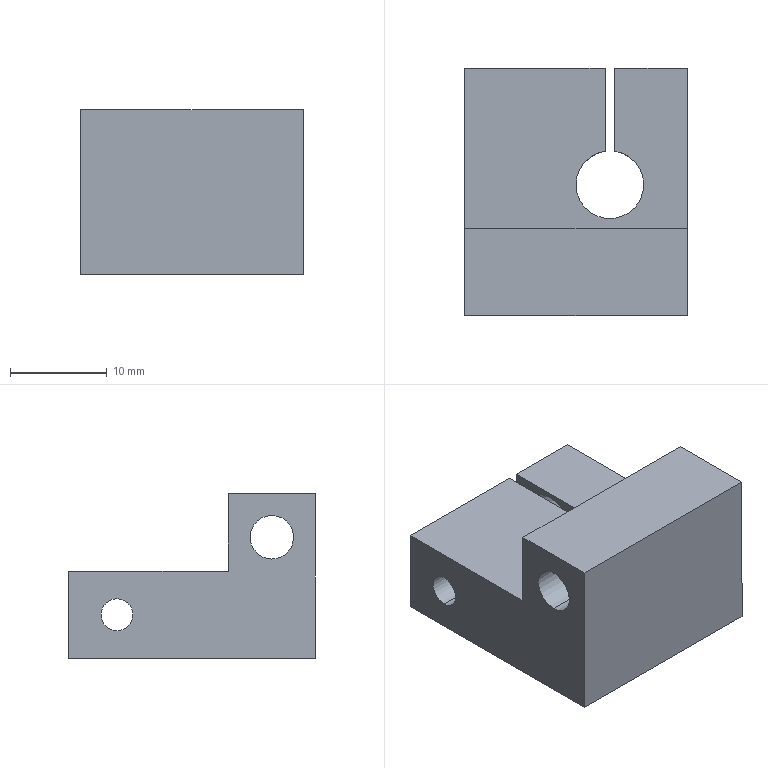Component | SolidWorks | AS-011-JG0137-1 | 1 solid | 26 faces | box 23 x 25.5 x 17 mm | volume 5301 mm3 | cylinder 13 | plane 13 | commonest cylinder face diameters 8 x4 7 x3 7.5 x2 4.5 x2 3.3 x2
STEP:
#1=COLOUR_RGB('',0.7922,0.8196,0.9333);
#2=FILL_AREA_STYLE_COLOUR('',#1);
#3=FILL_AREA_STYLE('',(#2));
#4=SURFACE_STYLE_FILL_AREA(#3);
#5=SURFACE_SIDE_STYLE('',(#4));
#6=SURFACE_STYLE_USAGE(.BOTH.,#5);
#7=PRESENTATION_STYLE_ASSIGNMENT((#6));
#8=CARTESIAN_POINT('',(-0.7283,-1.102,-1.476));
#9=VERTEX_POINT('',#8);
#10=CARTESIAN_POINT('',(-0.4528,-1.102,-1.476));
#11=VERTEX_POINT('',#10);
#12=CARTESIAN_POINT('',(-0.5906,-1.102,-1.476));
#13=DIRECTION('',(-0.,0.,1.));
#14=DIRECTION('',(1.,0.,0.));
#15=AXIS2_PLACEMENT_3D('',#12,#13,#14);
#16=CIRCLE('',#15,0.1378);
#17=EDGE_CURVE('',#9,#11,#16,.T.);
#18=ORIENTED_EDGE('',*,*,#17,.F.);
#19=CARTESIAN_POINT('',(-0.7283,-1.102,-1.122));
#20=VERTEX_POINT('',#19);
#21=CARTESIAN_POINT('',(-0.7283,-1.102,-1.476));
#22=DIRECTION('',(-0.,0.,1.));
#23=VECTOR('',#22,39.37);
#24=LINE('',#21,#23);
#25=EDGE_CURVE('',#9,#20,#24,.T.);
#26=ORIENTED_EDGE('',*,*,#25,.T.);
#27=CARTESIAN_POINT('',(-0.4528,-1.102,-1.122));
#28=VERTEX_POINT('',#27);
#29=CARTESIAN_POINT('',(-0.5906,-1.102,-1.122));
#30=DIRECTION('',(-0.,0.,1.));
#31=DIRECTION('',(1.,0.,0.));
#32=AXIS2_PLACEMENT_3D('',#29,#30,#31);
#33=CIRCLE('',#32,0.1378);
#34=EDGE_CURVE('',#20,#28,#33,.T.);
#35=ORIENTED_EDGE('',*,*,#34,.T.);
#36=CARTESIAN_POINT('',(-0.4528,-1.102,-1.476));
#37=DIRECTION('',(-0.,0.,1.));
#38=VECTOR('',#37,39.37);
#39=LINE('',#36,#38);
#40=EDGE_CURVE('',#11,#28,#39,.T.);
#41=ORIENTED_EDGE('',*,*,#40,.F.);
#42=EDGE_LOOP('',(#18,#26,#35,#41));
#43=FACE_OUTER_BOUND('',#42,.T.);
#44=CARTESIAN_POINT('',(-0.5906,-1.102,-1.476));
#45=DIRECTION('',(-0.,0.,1.));
#46=DIRECTION('',(1.,0.,0.));
#47=AXIS2_PLACEMENT_3D('',#44,#45,#46);
#48=CYLINDRICAL_SURFACE('',#47,0.1378);
#49=ADVANCED_FACE('',(#43),#48,.F.);
#50=CARTESIAN_POINT('',(-0.5709,-0.966,-1.476));
#51=VERTEX_POINT('',#50);
#52=CARTESIAN_POINT('',(-0.5906,-1.102,-1.476));
#53=DIRECTION('',(-0.,0.,1.));
#54=DIRECTION('',(1.,0.,0.));
#55=AXIS2_PLACEMENT_3D('',#52,#53,#54);
#56=CIRCLE('',#55,0.1378);
#57=EDGE_CURVE('',#11,#51,#56,.T.);
#58=ORIENTED_EDGE('',*,*,#57,.F.);
#59=ORIENTED_EDGE('',*,*,#40,.T.);
#60=CARTESIAN_POINT('',(-0.5709,-0.966,-1.122));
#61=VERTEX_POINT('',#60);
#62=CARTESIAN_POINT('',(-0.5906,-1.102,-1.122));
#63=DIRECTION('',(-0.,0.,1.));
#64=DIRECTION('',(1.,0.,0.));
#65=AXIS2_PLACEMENT_3D('',#62,#63,#64);
#66=CIRCLE('',#65,0.1378);
#67=EDGE_CURVE('',#28,#61,#66,.T.);
#68=ORIENTED_EDGE('',*,*,#67,.T.);
#69=CARTESIAN_POINT('',(-0.5709,-0.966,-1.226));
#70=VERTEX_POINT('',#69);
#71=CARTESIAN_POINT('',(-0.5709,-0.966,-1.476));
#72=DIRECTION('',(-0.,0.,1.));
#73=VECTOR('',#72,39.37);
#74=LINE('',#71,#73);
#75=EDGE_CURVE('',#70,#61,#74,.T.);
#76=ORIENTED_EDGE('',*,*,#75,.F.);
#77=CARTESIAN_POINT('',(-0.5709,-0.966,-1.373));
#78=VERTEX_POINT('',#77);
#79=CARTESIAN_POINT('',(-0.5709,-0.966,-1.373));
#80=CARTESIAN_POINT('',(-0.5629,-0.9671,-1.371));
#81=CARTESIAN_POINT('',(-0.5557,-0.9689,-1.367));
#82=CARTESIAN_POINT('',(-0.5426,-0.973,-1.358));
#83=CARTESIAN_POINT('',(-0.5371,-0.9752,-1.352));
#84=CARTESIAN_POINT('',(-0.5282,-0.9794,-1.339));
#85=CARTESIAN_POINT('',(-0.525,-0.9811,-1.331));
#86=CARTESIAN_POINT('',(-0.5206,-0.9836,-1.316));
#87=CARTESIAN_POINT('',(-0.5196,-0.9843,-1.307));
#88=CARTESIAN_POINT('',(-0.5196,-0.9843,-1.291));
#89=CARTESIAN_POINT('',(-0.5206,-0.9836,-1.283));
#90=CARTESIAN_POINT('',(-0.525,-0.9811,-1.267));
#91=CARTESIAN_POINT('',(-0.5282,-0.9794,-1.26));
#92=CARTESIAN_POINT('',(-0.5349,-0.9763,-1.25));
#93=CARTESIAN_POINT('',(-0.5374,-0.9752,-1.247));
#94=CARTESIAN_POINT('',(-0.5428,-0.9731,-1.241));
#95=CARTESIAN_POINT('',(-0.5458,-0.972,-1.238));
#96=CARTESIAN_POINT('',(-0.5523,-0.9699,-1.234));
#97=CARTESIAN_POINT('',(-0.5558,-0.969,-1.232));
#98=CARTESIAN_POINT('',(-0.5631,-0.9673,-1.228));
#99=CARTESIAN_POINT('',(-0.5669,-0.9666,-1.227));
#100=CARTESIAN_POINT('',(-0.5709,-0.966,-1.226));
#101=B_SPLINE_CURVE_WITH_KNOTS('',3,(#79,#80,#81,#82,#83,#84,#85,#86,#87,#88,#89,#90,#91,#92,#93,#94,#95,#96,#97,#98,#99,#100),.UNSPECIFIED.,.F.,.F.,(4,2,2,2,2,2,2,2,2,2,4),(0.,0.0006232,0.001246,0.00187,0.002493,0.003116,0.003739,0.004051,0.004363,0.004674,0.004986),.UNSPECIFIED.);
#102=EDGE_CURVE('',#78,#70,#101,.T.);
#103=ORIENTED_EDGE('',*,*,#102,.F.);
#104=CARTESIAN_POINT('',(-0.5709,-0.966,-1.476));
#105=DIRECTION('',(-0.,0.,1.));
#106=VECTOR('',#105,39.37);
#107=LINE('',#104,#106);
#108=EDGE_CURVE('',#51,#78,#107,.T.);
#109=ORIENTED_EDGE('',*,*,#108,.F.);
#110=EDGE_LOOP('',(#58,#59,#68,#76,#103,#109));
#111=FACE_OUTER_BOUND('',#110,.T.);
#112=CARTESIAN_POINT('',(-0.5906,-1.102,-1.476));
#113=DIRECTION('',(-0.,0.,1.));
#114=DIRECTION('',(1.,0.,0.));
#115=AXIS2_PLACEMENT_3D('',#112,#113,#114);
#116=CYLINDRICAL_SURFACE('',#115,0.1378);
#117=ADVANCED_FACE('',(#111),#116,.F.);
#118=CARTESIAN_POINT('',(-0.6693,-1.457,-0.8366));
#119=VERTEX_POINT('',#118);
#120=CARTESIAN_POINT('',(-0.6693,-1.457,-1.132));
#121=VERTEX_POINT('',#120);
#122=CARTESIAN_POINT('',(-0.6693,-1.457,-0.9843));
#123=DIRECTION('',(1.,0.,0.));
#124=DIRECTION('',(0.,0.,-1.));
#125=AXIS2_PLACEMENT_3D('',#122,#123,#124);
#126=CIRCLE('',#125,0.1476);
#127=EDGE_CURVE('',#119,#121,#126,.T.);
#128=ORIENTED_EDGE('',*,*,#127,.F.);
#129=CARTESIAN_POINT('',(-0.2756,-1.457,-0.8366));
#130=VERTEX_POINT('',#129);
#131=CARTESIAN_POINT('',(-0.6693,-1.457,-0.8366));
#132=DIRECTION('',(1.,0.,0.));
#133=VECTOR('',#132,39.37);
#134=LINE('',#131,#133);
#135=EDGE_CURVE('',#119,#130,#134,.T.);
#136=ORIENTED_EDGE('',*,*,#135,.T.);
#137=CARTESIAN_POINT('',(-0.2756,-1.457,-1.132));
#138=VERTEX_POINT('',#137);
#139=CARTESIAN_POINT('',(-0.2756,-1.457,-0.9843));
#140=DIRECTION('',(1.,0.,0.));
#141=DIRECTION('',(0.,0.,-1.));
#142=AXIS2_PLACEMENT_3D('',#139,#140,#141);
#143=CIRCLE('',#142,0.1476);
#144=EDGE_CURVE('',#130,#138,#143,.T.);
#145=ORIENTED_EDGE('',*,*,#144,.T.);
#146=CARTESIAN_POINT('',(-0.6693,-1.457,-1.132));
#147=DIRECTION('',(1.,0.,0.));
#148=VECTOR('',#147,39.37);
#149=LINE('',#146,#148);
#150=EDGE_CURVE('',#121,#138,#149,.T.);
#151=ORIENTED_EDGE('',*,*,#150,.F.);
#152=EDGE_LOOP('',(#128,#136,#145,#151));
#153=FACE_OUTER_BOUND('',#152,.T.);
#154=CARTESIAN_POINT('',(-0.6693,-1.457,-0.9843));
#155=DIRECTION('',(1.,0.,0.));
#156=DIRECTION('',(0.,0.,-1.));
#157=AXIS2_PLACEMENT_3D('',#154,#155,#156);
#158=CYLINDRICAL_SURFACE('',#157,0.1476);
#159=ADVANCED_FACE('',(#153),#158,.F.);
#160=CARTESIAN_POINT('',(-0.5709,-0.8268,-1.142));
#161=VERTEX_POINT('',#160);
#162=CARTESIAN_POINT('',(-0.5709,-0.8268,-1.299));
#163=DIRECTION('',(1.,0.,0.));
#164=DIRECTION('',(0.,0.,1.));
#165=AXIS2_PLACEMENT_3D('',#162,#163,#164);
#166=CIRCLE('',#165,0.1575);
#167=EDGE_CURVE('',#161,#70,#166,.T.);
#168=ORIENTED_EDGE('',*,*,#167,.F.);
#169=CARTESIAN_POINT('',(-0.2756,-0.8268,-1.142));
#170=VERTEX_POINT('',#169);
#171=CARTESIAN_POINT('',(-0.6693,-0.8268,-1.142));
#172=DIRECTION('',(1.,0.,0.));
#173=VECTOR('',#172,39.37);
#174=LINE('',#171,#173);
#175=EDGE_CURVE('',#161,#170,#174,.T.);
#176=ORIENTED_EDGE('',*,*,#175,.T.);
#177=CARTESIAN_POINT('',(-0.2756,-0.8268,-1.457));
#178=VERTEX_POINT('',#177);
#179=CARTESIAN_POINT('',(-0.2756,-0.8268,-1.299));
#180=DIRECTION('',(1.,0.,0.));
#181=DIRECTION('',(0.,-0.,-1.));
#182=AXIS2_PLACEMENT_3D('',#179,#180,#181);
#183=CIRCLE('',#182,0.1575);
#184=EDGE_CURVE('',#170,#178,#183,.T.);
#185=ORIENTED_EDGE('',*,*,#184,.T.);
#186=CARTESIAN_POINT('',(-0.5709,-0.8268,-1.457));
#187=VERTEX_POINT('',#186);
#188=CARTESIAN_POINT('',(-0.6693,-0.8268,-1.457));
#189=DIRECTION('',(1.,0.,0.));
#190=VECTOR('',#189,39.37);
#191=LINE('',#188,#190);
#192=EDGE_CURVE('',#187,#178,#191,.T.);
#193=ORIENTED_EDGE('',*,*,#192,.F.);
#194=CARTESIAN_POINT('',(-0.5709,-0.8268,-1.299));
#195=DIRECTION('',(1.,0.,0.));
#196=DIRECTION('',(0.,-0.,1.));
#197=AXIS2_PLACEMENT_3D('',#194,#195,#196);
#198=CIRCLE('',#197,0.1575);
#199=EDGE_CURVE('',#78,#187,#198,.T.);
#200=ORIENTED_EDGE('',*,*,#199,.F.);
#201=ORIENTED_EDGE('',*,*,#102,.T.);
#202=EDGE_LOOP('',(#168,#176,#185,#193,#200,#201));
#203=FACE_OUTER_BOUND('',#202,.T.);
#204=CARTESIAN_POINT('',(-0.6693,-0.8268,-1.299));
#205=DIRECTION('',(1.,0.,0.));
#206=DIRECTION('',(0.,-0.,-1.));
#207=AXIS2_PLACEMENT_3D('',#204,#205,#206);
#208=CYLINDRICAL_SURFACE('',#207,0.1575);
#209=ADVANCED_FACE('',(#203),#208,.F.);
#210=CARTESIAN_POINT('',(-1.181,-1.457,-0.8957));
#211=VERTEX_POINT('',#210);
#212=CARTESIAN_POINT('',(-1.181,-1.457,-1.073));
#213=VERTEX_POINT('',#212);
#214=CARTESIAN_POINT('',(-1.181,-1.457,-0.9843));
#215=DIRECTION('',(1.,0.,0.));
#216=DIRECTION('',(0.,0.,-1.));
#217=AXIS2_PLACEMENT_3D('',#214,#215,#216);
#218=CIRCLE('',#217,0.08858);
#219=EDGE_CURVE('',#211,#213,#218,.T.);
#220=ORIENTED_EDGE('',*,*,#219,.F.);
#221=CARTESIAN_POINT('',(-0.6693,-1.457,-0.8957));
#222=VERTEX_POINT('',#221);
#223=CARTESIAN_POINT('',(-1.181,-1.457,-0.8957));
#224=DIRECTION('',(1.,0.,0.));
#225=VECTOR('',#224,39.37);
#226=LINE('',#223,#225);
#227=EDGE_CURVE('',#211,#222,#226,.T.);
#228=ORIENTED_EDGE('',*,*,#227,.T.);
#229=CARTESIAN_POINT('',(-0.6693,-1.457,-1.073));
#230=VERTEX_POINT('',#229);
#231=CARTESIAN_POINT('',(-0.6693,-1.457,-0.9843));
#232=DIRECTION('',(1.,0.,0.));
#233=DIRECTION('',(0.,0.,-1.));
#234=AXIS2_PLACEMENT_3D('',#231,#232,#233);
#235=CIRCLE('',#234,0.08858);
#236=EDGE_CURVE('',#222,#230,#235,.T.);
#237=ORIENTED_EDGE('',*,*,#236,.T.);
#238=CARTESIAN_POINT('',(-1.181,-1.457,-1.073));
#239=DIRECTION('',(1.,0.,0.));
#240=VECTOR('',#239,39.37);
#241=LINE('',#238,#240);
#242=EDGE_CURVE('',#213,#230,#241,.T.);
#243=ORIENTED_EDGE('',*,*,#242,.F.);
#244=EDGE_LOOP('',(#220,#228,#237,#243));
#245=FACE_OUTER_BOUND('',#244,.T.);
#246=CARTESIAN_POINT('',(-1.181,-1.457,-0.9843));
#247=DIRECTION('',(1.,0.,0.));
#248=DIRECTION('',(0.,0.,-1.));
#249=AXIS2_PLACEMENT_3D('',#246,#247,#248);
#250=CYLINDRICAL_SURFACE('',#249,0.08858);
#251=ADVANCED_FACE('',(#245),#250,.F.);
#252=CARTESIAN_POINT('',(-1.181,-0.8268,-1.234));
#253=VERTEX_POINT('',#252);
#254=CARTESIAN_POINT('',(-1.181,-0.8268,-1.364));
#255=VERTEX_POINT('',#254);
#256=CARTESIAN_POINT('',(-1.181,-0.8268,-1.299));
#257=DIRECTION('',(1.,0.,0.));
#258=DIRECTION('',(0.,0.,-1.));
#259=AXIS2_PLACEMENT_3D('',#256,#257,#258);
#260=CIRCLE('',#259,0.06496);
#261=EDGE_CURVE('',#253,#255,#260,.T.);
#262=ORIENTED_EDGE('',*,*,#261,.F.);
#263=CARTESIAN_POINT('',(-0.6693,-0.8268,-1.234));
#264=VERTEX_POINT('',#263);
#265=CARTESIAN_POINT('',(-1.181,-0.8268,-1.234));
#266=DIRECTION('',(1.,0.,0.));
#267=VECTOR('',#266,39.37);
#268=LINE('',#265,#267);
#269=EDGE_CURVE('',#253,#264,#268,.T.);
#270=ORIENTED_EDGE('',*,*,#269,.T.);
#271=CARTESIAN_POINT('',(-0.6693,-0.8268,-1.364));
#272=VERTEX_POINT('',#271);
#273=CARTESIAN_POINT('',(-0.6693,-0.8268,-1.299));
#274=DIRECTION('',(1.,0.,0.));
#275=DIRECTION('',(0.,0.,-1.));
#276=AXIS2_PLACEMENT_3D('',#273,#274,#275);
#277=CIRCLE('',#276,0.06496);
#278=EDGE_CURVE('',#264,#272,#277,.T.);
#279=ORIENTED_EDGE('',*,*,#278,.T.);
#280=CARTESIAN_POINT('',(-1.181,-0.8268,-1.364));
#281=DIRECTION('',(1.,0.,0.));
#282=VECTOR('',#281,39.37);
#283=LINE('',#280,#282);
#284=EDGE_CURVE('',#255,#272,#283,.T.);
#285=ORIENTED_EDGE('',*,*,#284,.F.);
#286=EDGE_LOOP('',(#262,#270,#279,#285));
#287=FACE_OUTER_BOUND('',#286,.T.);
#288=CARTESIAN_POINT('',(-1.181,-0.8268,-1.299));
#289=DIRECTION('',(1.,0.,0.));
#290=DIRECTION('',(0.,0.,-1.));
#291=AXIS2_PLACEMENT_3D('',#288,#289,#290);
#292=CYLINDRICAL_SURFACE('',#291,0.06496);
#293=ADVANCED_FACE('',(#287),#292,.F.);
#294=CARTESIAN_POINT('',(-0.6693,-0.8268,-1.142));
#295=VERTEX_POINT('',#294);
#296=CARTESIAN_POINT('',(-0.6693,-0.8268,-1.457));
#297=VERTEX_POINT('',#296);
#298=CARTESIAN_POINT('',(-0.6693,-0.8268,-1.299));
#299=DIRECTION('',(1.,0.,0.));
#300=DIRECTION('',(0.,-0.,-1.));
#301=AXIS2_PLACEMENT_3D('',#298,#299,#300);
#302=CIRCLE('',#301,0.1575);
#303=EDGE_CURVE('',#295,#297,#302,.T.);
#304=ORIENTED_EDGE('',*,*,#303,.F.);
#305=CARTESIAN_POINT('',(-0.6102,-0.8268,-1.142));
#306=VERTEX_POINT('',#305);
#307=CARTESIAN_POINT('',(-0.6693,-0.8268,-1.142));
#308=DIRECTION('',(1.,0.,0.));
#309=VECTOR('',#308,39.37);
#310=LINE('',#307,#309);
#311=EDGE_CURVE('',#295,#306,#310,.T.);
#312=ORIENTED_EDGE('',*,*,#311,.T.);
#313=CARTESIAN_POINT('',(-0.6102,-0.966,-1.226));
#314=VERTEX_POINT('',#313);
#315=CARTESIAN_POINT('',(-0.6102,-0.8268,-1.299));
#316=DIRECTION('',(1.,0.,0.));
#317=DIRECTION('',(0.,0.,1.));
#318=AXIS2_PLACEMENT_3D('',#315,#316,#317);
#319=CIRCLE('',#318,0.1575);
#320=EDGE_CURVE('',#306,#314,#319,.T.);
#321=ORIENTED_EDGE('',*,*,#320,.T.);
#322=CARTESIAN_POINT('',(-0.6102,-0.966,-1.373));
#323=VERTEX_POINT('',#322);
#324=CARTESIAN_POINT('',(-0.6102,-0.966,-1.226));
#325=CARTESIAN_POINT('',(-0.6182,-0.9671,-1.228));
#326=CARTESIAN_POINT('',(-0.6254,-0.9689,-1.231));
#327=CARTESIAN_POINT('',(-0.6385,-0.973,-1.241));
#328=CARTESIAN_POINT('',(-0.644,-0.9752,-1.246));
#329=CARTESIAN_POINT('',(-0.6529,-0.9794,-1.26));
#330=CARTESIAN_POINT('',(-0.6561,-0.9811,-1.267));
#331=CARTESIAN_POINT('',(-0.6605,-0.9836,-1.283));
#332=CARTESIAN_POINT('',(-0.6615,-0.9843,-1.291));
#333=CARTESIAN_POINT('',(-0.6615,-0.9843,-1.308));
#334=CARTESIAN_POINT('',(-0.6605,-0.9836,-1.316));
#335=CARTESIAN_POINT('',(-0.6561,-0.9811,-1.331));
#336=CARTESIAN_POINT('',(-0.6529,-0.9794,-1.339));
#337=CARTESIAN_POINT('',(-0.6463,-0.9763,-1.349));
#338=CARTESIAN_POINT('',(-0.6437,-0.9752,-1.352));
#339=CARTESIAN_POINT('',(-0.6383,-0.9731,-1.358));
#340=CARTESIAN_POINT('',(-0.6353,-0.972,-1.36));
#341=CARTESIAN_POINT('',(-0.6288,-0.9699,-1.365));
#342=CARTESIAN_POINT('',(-0.6253,-0.969,-1.367));
#343=CARTESIAN_POINT('',(-0.618,-0.9673,-1.37));
#344=CARTESIAN_POINT('',(-0.6142,-0.9666,-1.372));
#345=CARTESIAN_POINT('',(-0.6102,-0.966,-1.373));
#346=B_SPLINE_CURVE_WITH_KNOTS('',3,(#324,#325,#326,#327,#328,#329,#330,#331,#332,#333,#334,#335,#336,#337,#338,#339,#340,#341,#342,#343,#344,#345),.UNSPECIFIED.,.F.,.F.,(4,2,2,2,2,2,2,2,2,2,4),(0.,0.0006232,0.001246,0.00187,0.002493,0.003116,0.003739,0.004051,0.004363,0.004674,0.004986),.UNSPECIFIED.);
#347=EDGE_CURVE('',#314,#323,#346,.T.);
#348=ORIENTED_EDGE('',*,*,#347,.T.);
#349=CARTESIAN_POINT('',(-0.6102,-0.8268,-1.457));
#350=VERTEX_POINT('',#349);
#351=CARTESIAN_POINT('',(-0.6102,-0.8268,-1.299));
#352=DIRECTION('',(1.,0.,0.));
#353=DIRECTION('',(0.,-0.,1.));
#354=AXIS2_PLACEMENT_3D('',#351,#352,#353);
#355=CIRCLE('',#354,0.1575);
#356=EDGE_CURVE('',#323,#350,#355,.T.);
#357=ORIENTED_EDGE('',*,*,#356,.T.);
#358=CARTESIAN_POINT('',(-0.6693,-0.8268,-1.457));
#359=DIRECTION('',(1.,0.,0.));
#360=VECTOR('',#359,39.37);
#361=LINE('',#358,#360);
#362=EDGE_CURVE('',#297,#350,#361,.T.);
#363=ORIENTED_EDGE('',*,*,#362,.F.);
#364=EDGE_LOOP('',(#304,#312,#321,#348,#357,#363));
#365=FACE_OUTER_BOUND('',#364,.T.);
#366=CARTESIAN_POINT('',(-0.6693,-0.8268,-1.299));
#367=DIRECTION('',(1.,0.,0.));
#368=DIRECTION('',(0.,-0.,-1.));
#369=AXIS2_PLACEMENT_3D('',#366,#367,#368);
#370=CYLINDRICAL_SURFACE('',#369,0.1575);
#371=ADVANCED_FACE('',(#365),#370,.F.);
#372=CARTESIAN_POINT('',(-0.5709,-0.6299,-1.476));
#373=VERTEX_POINT('',#372);
#374=CARTESIAN_POINT('',(-0.5709,-0.6299,-1.122));
#375=VERTEX_POINT('',#374);
#376=CARTESIAN_POINT('',(-0.5709,-0.6299,-1.476));
#377=DIRECTION('',(-0.,0.,1.));
#378=VECTOR('',#377,39.37);
#379=LINE('',#376,#378);
#380=EDGE_CURVE('',#373,#375,#379,.T.);
#381=ORIENTED_EDGE('',*,*,#380,.T.);
#382=CARTESIAN_POINT('',(-0.2756,-0.6299,-1.122));
#383=VERTEX_POINT('',#382);
#384=CARTESIAN_POINT('',(-1.181,-0.6299,-1.122));
#385=DIRECTION('',(1.,0.,0.));
#386=VECTOR('',#385,39.37);
#387=LINE('',#384,#386);
#388=EDGE_CURVE('',#375,#383,#387,.T.);
#389=ORIENTED_EDGE('',*,*,#388,.T.);
#390=CARTESIAN_POINT('',(-0.2756,-0.6299,-1.476));
#391=VERTEX_POINT('',#390);
#392=CARTESIAN_POINT('',(-0.2756,-0.6299,-1.122));
#393=DIRECTION('',(0.,-0.,-1.));
#394=VECTOR('',#393,39.37);
#395=LINE('',#392,#394);
#396=EDGE_CURVE('',#383,#391,#395,.T.);
#397=ORIENTED_EDGE('',*,*,#396,.T.);
#398=CARTESIAN_POINT('',(-1.181,-0.6299,-1.476));
#399=DIRECTION('',(1.,0.,0.));
#400=VECTOR('',#399,39.37);
#401=LINE('',#398,#400);
#402=EDGE_CURVE('',#373,#391,#401,.T.);
#403=ORIENTED_EDGE('',*,*,#402,.F.);
#404=EDGE_LOOP('',(#381,#389,#397,#403));
#405=FACE_OUTER_BOUND('',#404,.T.);
#406=CARTESIAN_POINT('',(-1.181,-0.6299,-1.122));
#407=DIRECTION('',(0.,-1.,0.));
#408=DIRECTION('',(-1.,-0.,-0.));
#409=AXIS2_PLACEMENT_3D('',#406,#407,#408);
#410=PLANE('',#409);
#411=ADVANCED_FACE('',(#405),#410,.F.);
#412=ORIENTED_EDGE('',*,*,#311,.F.);
#413=CARTESIAN_POINT('',(-0.6693,-0.8268,-1.299));
#414=DIRECTION('',(1.,0.,0.));
#415=DIRECTION('',(0.,-0.,-1.));
#416=AXIS2_PLACEMENT_3D('',#413,#414,#415);
#417=CIRCLE('',#416,0.1575);
#418=EDGE_CURVE('',#297,#295,#417,.T.);
#419=ORIENTED_EDGE('',*,*,#418,.F.);
#420=ORIENTED_EDGE('',*,*,#362,.T.);
#421=CARTESIAN_POINT('',(-0.6102,-0.8268,-1.299));
#422=DIRECTION('',(1.,0.,0.));
#423=DIRECTION('',(0.,0.,1.));
#424=AXIS2_PLACEMENT_3D('',#421,#422,#423);
#425=CIRCLE('',#424,0.1575);
#426=EDGE_CURVE('',#350,#306,#425,.T.);
#427=ORIENTED_EDGE('',*,*,#426,.T.);
#428=EDGE_LOOP('',(#412,#419,#420,#427));
#429=FACE_OUTER_BOUND('',#428,.T.);
#430=CARTESIAN_POINT('',(-0.6693,-0.8268,-1.299));
#431=DIRECTION('',(1.,0.,0.));
#432=DIRECTION('',(0.,-0.,-1.));
#433=AXIS2_PLACEMENT_3D('',#430,#431,#432);
#434=CYLINDRICAL_SURFACE('',#433,0.1575);
#435=ADVANCED_FACE('',(#429),#434,.F.);
#436=ORIENTED_EDGE('',*,*,#269,.F.);
#437=CARTESIAN_POINT('',(-1.181,-0.8268,-1.299));
#438=DIRECTION('',(1.,0.,0.));
#439=DIRECTION('',(0.,0.,-1.));
#440=AXIS2_PLACEMENT_3D('',#437,#438,#439);
#441=CIRCLE('',#440,0.06496);
#442=EDGE_CURVE('',#255,#253,#441,.T.);
#443=ORIENTED_EDGE('',*,*,#442,.F.);
#444=ORIENTED_EDGE('',*,*,#284,.T.);
#445=CARTESIAN_POINT('',(-0.6693,-0.8268,-1.299));
#446=DIRECTION('',(1.,0.,0.));
#447=DIRECTION('',(0.,0.,-1.));
#448=AXIS2_PLACEMENT_3D('',#445,#446,#447);
#449=CIRCLE('',#448,0.06496);
#450=EDGE_CURVE('',#272,#264,#449,.T.);
#451=ORIENTED_EDGE('',*,*,#450,.T.);
#452=EDGE_LOOP('',(#436,#443,#444,#451));
#453=FACE_OUTER_BOUND('',#452,.T.);
#454=CARTESIAN_POINT('',(-1.181,-0.8268,-1.299));
#455=DIRECTION('',(1.,0.,0.));
#456=DIRECTION('',(0.,0.,-1.));
#457=AXIS2_PLACEMENT_3D('',#454,#455,#456);
#458=CYLINDRICAL_SURFACE('',#457,0.06496);
#459=ADVANCED_FACE('',(#453),#458,.F.);
#460=ORIENTED_EDGE('',*,*,#227,.F.);
#461=CARTESIAN_POINT('',(-1.181,-1.457,-0.9843));
#462=DIRECTION('',(1.,0.,0.));
#463=DIRECTION('',(0.,0.,-1.));
#464=AXIS2_PLACEMENT_3D('',#461,#462,#463);
#465=CIRCLE('',#464,0.08858);
#466=EDGE_CURVE('',#213,#211,#465,.T.);
#467=ORIENTED_EDGE('',*,*,#466,.F.);
#468=ORIENTED_EDGE('',*,*,#242,.T.);
#469=CARTESIAN_POINT('',(-0.6693,-1.457,-0.9843));
#470=DIRECTION('',(1.,0.,0.));
#471=DIRECTION('',(0.,0.,-1.));
#472=AXIS2_PLACEMENT_3D('',#469,#470,#471);
#473=CIRCLE('',#472,0.08858);
#474=EDGE_CURVE('',#230,#222,#473,.T.);
#475=ORIENTED_EDGE('',*,*,#474,.T.);
#476=EDGE_LOOP('',(#460,#467,#468,#475));
#477=FACE_OUTER_BOUND('',#476,.T.);
#478=CARTESIAN_POINT('',(-1.181,-1.457,-0.9843));
#479=DIRECTION('',(1.,0.,0.));
#480=DIRECTION('',(0.,0.,-1.));
#481=AXIS2_PLACEMENT_3D('',#478,#479,#480);
#482=CYLINDRICAL_SURFACE('',#481,0.08858);
#483=ADVANCED_FACE('',(#477),#482,.F.);
#484=CARTESIAN_POINT('',(-1.181,-0.6299,-1.476));
#485=VERTEX_POINT('',#484);
#486=CARTESIAN_POINT('',(-0.6102,-0.6299,-1.476));
#487=VERTEX_POINT('',#486);
#488=CARTESIAN_POINT('',(-1.181,-0.6299,-1.476));
#489=DIRECTION('',(1.,0.,0.));
#490=VECTOR('',#489,39.37);
#491=LINE('',#488,#490);
#492=EDGE_CURVE('',#485,#487,#491,.T.);
#493=ORIENTED_EDGE('',*,*,#492,.T.);
#494=CARTESIAN_POINT('',(-0.6102,-0.966,-1.476));
#495=VERTEX_POINT('',#494);
#496=CARTESIAN_POINT('',(-0.6102,-0.6299,-1.476));
#497=DIRECTION('',(0.,-1.,0.));
#498=VECTOR('',#497,39.37);
#499=LINE('',#496,#498);
#500=EDGE_CURVE('',#487,#495,#499,.T.);
#501=ORIENTED_EDGE('',*,*,#500,.T.);
#502=CARTESIAN_POINT('',(-0.5906,-1.102,-1.476));
#503=DIRECTION('',(-0.,0.,1.));
#504=DIRECTION('',(1.,0.,0.));
#505=AXIS2_PLACEMENT_3D('',#502,#503,#504);
#506=CIRCLE('',#505,0.1378);
#507=EDGE_CURVE('',#495,#9,#506,.T.);
#508=ORIENTED_EDGE('',*,*,#507,.T.);
#509=ORIENTED_EDGE('',*,*,#17,.T.);
#510=ORIENTED_EDGE('',*,*,#57,.T.);
#511=CARTESIAN_POINT('',(-0.5709,-0.6299,-1.476));
#512=DIRECTION('',(0.,-1.,0.));
#513=VECTOR('',#512,39.37);
#514=LINE('',#511,#513);
#515=EDGE_CURVE('',#373,#51,#514,.T.);
#516=ORIENTED_EDGE('',*,*,#515,.F.);
#517=ORIENTED_EDGE('',*,*,#402,.T.);
#518=CARTESIAN_POINT('',(-0.2756,-1.634,-1.476));
#519=VERTEX_POINT('',#518);
#520=CARTESIAN_POINT('',(-0.2756,-0.6299,-1.476));
#521=DIRECTION('',(0.,-1.,0.));
#522=VECTOR('',#521,39.37);
#523=LINE('',#520,#522);
#524=EDGE_CURVE('',#391,#519,#523,.T.);
#525=ORIENTED_EDGE('',*,*,#524,.T.);
#526=CARTESIAN_POINT('',(-1.181,-1.634,-1.476));
#527=VERTEX_POINT('',#526);
#528=CARTESIAN_POINT('',(-1.181,-1.634,-1.476));
#529=DIRECTION('',(1.,0.,0.));
#530=VECTOR('',#529,39.37);
#531=LINE('',#528,#530);
#532=EDGE_CURVE('',#527,#519,#531,.T.);
#533=ORIENTED_EDGE('',*,*,#532,.F.);
#534=CARTESIAN_POINT('',(-1.181,-0.6299,-1.476));
#535=DIRECTION('',(0.,-1.,0.));
#536=VECTOR('',#535,39.37);
#537=LINE('',#534,#536);
#538=EDGE_CURVE('',#485,#527,#537,.T.);
#539=ORIENTED_EDGE('',*,*,#538,.F.);
#540=EDGE_LOOP('',(#493,#501,#508,#509,#510,#516,#517,#525,#533,#539));
#541=FACE_OUTER_BOUND('',#540,.T.);
#542=CARTESIAN_POINT('',(-1.181,-0.6299,-1.476));
#543=DIRECTION('',(-0.,0.,1.));
#544=DIRECTION('',(1.,0.,0.));
#545=AXIS2_PLACEMENT_3D('',#542,#543,#544);
#546=PLANE('',#545);
#547=ADVANCED_FACE('',(#541),#546,.F.);
#548=CARTESIAN_POINT('',(-0.2756,-1.634,-0.8071));
#549=VERTEX_POINT('',#548);
#550=CARTESIAN_POINT('',(-0.2756,-1.634,-0.8071));
#551=DIRECTION('',(0.,-0.,-1.));
#552=VECTOR('',#551,39.37);
#553=LINE('',#550,#552);
#554=EDGE_CURVE('',#549,#519,#553,.T.);
#555=ORIENTED_EDGE('',*,*,#554,.F.);
#556=CARTESIAN_POINT('',(-1.181,-1.634,-0.8071));
#557=VERTEX_POINT('',#556);
#558=CARTESIAN_POINT('',(-1.181,-1.634,-0.8071));
#559=DIRECTION('',(1.,0.,0.));
#560=VECTOR('',#559,39.37);
#561=LINE('',#558,#560);
#562=EDGE_CURVE('',#557,#549,#561,.T.);
#563=ORIENTED_EDGE('',*,*,#562,.F.);
#564=CARTESIAN_POINT('',(-1.181,-1.634,-0.8071));
#565=DIRECTION('',(0.,-0.,-1.));
#566=VECTOR('',#565,39.37);
#567=LINE('',#564,#566);
#568=EDGE_CURVE('',#557,#527,#567,.T.);
#569=ORIENTED_EDGE('',*,*,#568,.T.);
#570=ORIENTED_EDGE('',*,*,#532,.T.);
#571=EDGE_LOOP('',(#555,#563,#569,#570));
#572=FACE_OUTER_BOUND('',#571,.T.);
#573=CARTESIAN_POINT('',(-1.181,-1.634,-0.8071));
#574=DIRECTION('',(0.,-1.,0.));
#575=DIRECTION('',(-1.,-0.,-0.));
#576=AXIS2_PLACEMENT_3D('',#573,#574,#575);
#577=PLANE('',#576);
#578=ADVANCED_FACE('',(#572),#577,.T.);
#579=CARTESIAN_POINT('',(-0.2756,-1.28,-0.8071));
#580=VERTEX_POINT('',#579);
#581=CARTESIAN_POINT('',(-0.2756,-1.28,-0.8071));
#582=DIRECTION('',(0.,-1.,0.));
#583=VECTOR('',#582,39.37);
#584=LINE('',#581,#583);
#585=EDGE_CURVE('',#580,#549,#584,.T.);
#586=ORIENTED_EDGE('',*,*,#585,.F.);
#587=CARTESIAN_POINT('',(-1.181,-1.28,-0.8071));
#588=VERTEX_POINT('',#587);
#589=CARTESIAN_POINT('',(-1.181,-1.28,-0.8071));
#590=DIRECTION('',(1.,0.,0.));
#591=VECTOR('',#590,39.37);
#592=LINE('',#589,#591);
#593=EDGE_CURVE('',#588,#580,#592,.T.);
#594=ORIENTED_EDGE('',*,*,#593,.F.);
#595=CARTESIAN_POINT('',(-1.181,-1.28,-0.8071));
#596=DIRECTION('',(0.,-1.,0.));
#597=VECTOR('',#596,39.37);
#598=LINE('',#595,#597);
#599=EDGE_CURVE('',#588,#557,#598,.T.);
#600=ORIENTED_EDGE('',*,*,#599,.T.);
#601=ORIENTED_EDGE('',*,*,#562,.T.);
#602=EDGE_LOOP('',(#586,#594,#600,#601));
#603=FACE_OUTER_BOUND('',#602,.T.);
#604=CARTESIAN_POINT('',(-1.181,-1.28,-0.8071));
#605=DIRECTION('',(-0.,0.,1.));
#606=DIRECTION('',(1.,0.,0.));
#607=AXIS2_PLACEMENT_3D('',#604,#605,#606);
#608=PLANE('',#607);
#609=ADVANCED_FACE('',(#603),#608,.T.);
#610=CARTESIAN_POINT('',(-0.2756,-1.28,-1.122));
#611=VERTEX_POINT('',#610);
#612=CARTESIAN_POINT('',(-0.2756,-1.28,-0.8071));
#613=DIRECTION('',(0.,-0.,-1.));
#614=VECTOR('',#613,39.37);
#615=LINE('',#612,#614);
#616=EDGE_CURVE('',#580,#611,#615,.T.);
#617=ORIENTED_EDGE('',*,*,#616,.T.);
#618=CARTESIAN_POINT('',(-1.181,-1.28,-1.122));
#619=VERTEX_POINT('',#618);
#620=CARTESIAN_POINT('',(-1.181,-1.28,-1.122));
#621=DIRECTION('',(1.,0.,0.));
#622=VECTOR('',#621,39.37);
#623=LINE('',#620,#622);
#624=EDGE_CURVE('',#619,#611,#623,.T.);
#625=ORIENTED_EDGE('',*,*,#624,.F.);
#626=CARTESIAN_POINT('',(-1.181,-1.28,-0.8071));
#627=DIRECTION('',(0.,-0.,-1.));
#628=VECTOR('',#627,39.37);
#629=LINE('',#626,#628);
#630=EDGE_CURVE('',#588,#619,#629,.T.);
#631=ORIENTED_EDGE('',*,*,#630,.F.);
#632=ORIENTED_EDGE('',*,*,#593,.T.);
#633=EDGE_LOOP('',(#617,#625,#631,#632));
#634=FACE_OUTER_BOUND('',#633,.T.);
#635=CARTESIAN_POINT('',(-1.181,-1.28,-0.8071));
#636=DIRECTION('',(0.,-1.,0.));
#637=DIRECTION('',(-1.,-0.,-0.));
#638=AXIS2_PLACEMENT_3D('',#635,#636,#637);
#639=PLANE('',#638);
#640=ADVANCED_FACE('',(#634),#639,.F.);
#641=CARTESIAN_POINT('',(-0.6102,-0.6299,-1.122));
#642=VERTEX_POINT('',#641);
#643=CARTESIAN_POINT('',(-0.6102,-0.966,-1.122));
#644=VERTEX_POINT('',#643);
#645=CARTESIAN_POINT('',(-0.6102,-0.6299,-1.122));
#646=DIRECTION('',(0.,-1.,0.));
#647=VECTOR('',#646,39.37);
#648=LINE('',#645,#647);
#649=EDGE_CURVE('',#642,#644,#648,.T.);
#650=ORIENTED_EDGE('',*,*,#649,.F.);
#651=CARTESIAN_POINT('',(-1.181,-0.6299,-1.122));
#652=VERTEX_POINT('',#651);
#653=CARTESIAN_POINT('',(-1.181,-0.6299,-1.122));
#654=DIRECTION('',(1.,0.,0.));
#655=VECTOR('',#654,39.37);
#656=LINE('',#653,#655);
#657=EDGE_CURVE('',#652,#642,#656,.T.);
#658=ORIENTED_EDGE('',*,*,#657,.F.);
#659=CARTESIAN_POINT('',(-1.181,-0.6299,-1.122));
#660=DIRECTION('',(0.,-1.,0.));
#661=VECTOR('',#660,39.37);
#662=LINE('',#659,#661);
#663=EDGE_CURVE('',#652,#619,#662,.T.);
#664=ORIENTED_EDGE('',*,*,#663,.T.);
#665=ORIENTED_EDGE('',*,*,#624,.T.);
#666=CARTESIAN_POINT('',(-0.2756,-0.6299,-1.122));
#667=DIRECTION('',(0.,-1.,0.));
#668=VECTOR('',#667,39.37);
#669=LINE('',#666,#668);
#670=EDGE_CURVE('',#383,#611,#669,.T.);
#671=ORIENTED_EDGE('',*,*,#670,.F.);
#672=ORIENTED_EDGE('',*,*,#388,.F.);
#673=CARTESIAN_POINT('',(-0.5709,-0.6299,-1.122));
#674=DIRECTION('',(0.,-1.,0.));
#675=VECTOR('',#674,39.37);
#676=LINE('',#673,#675);
#677=EDGE_CURVE('',#375,#61,#676,.T.);
#678=ORIENTED_EDGE('',*,*,#677,.T.);
#679=ORIENTED_EDGE('',*,*,#67,.F.);
#680=ORIENTED_EDGE('',*,*,#34,.F.);
#681=CARTESIAN_POINT('',(-0.5906,-1.102,-1.122));
#682=DIRECTION('',(-0.,0.,1.));
#683=DIRECTION('',(1.,0.,0.));
#684=AXIS2_PLACEMENT_3D('',#681,#682,#683);
#685=CIRCLE('',#684,0.1378);
#686=EDGE_CURVE('',#644,#20,#685,.T.);
#687=ORIENTED_EDGE('',*,*,#686,.F.);
#688=EDGE_LOOP('',(#650,#658,#664,#665,#671,#672,#678,#679,#680,#687));
#689=FACE_OUTER_BOUND('',#688,.T.);
#690=CARTESIAN_POINT('',(-1.181,-0.6299,-1.122));
#691=DIRECTION('',(-0.,0.,1.));
#692=DIRECTION('',(1.,0.,0.));
#693=AXIS2_PLACEMENT_3D('',#690,#691,#692);
#694=PLANE('',#693);
#695=ADVANCED_FACE('',(#689),#694,.T.);
#696=ORIENTED_EDGE('',*,*,#657,.T.);
#697=CARTESIAN_POINT('',(-0.6102,-0.6299,-1.476));
#698=DIRECTION('',(-0.,0.,1.));
#699=VECTOR('',#698,39.37);
#700=LINE('',#697,#699);
#701=EDGE_CURVE('',#487,#642,#700,.T.);
#702=ORIENTED_EDGE('',*,*,#701,.F.);
#703=ORIENTED_EDGE('',*,*,#492,.F.);
#704=CARTESIAN_POINT('',(-1.181,-0.6299,-1.122));
#705=DIRECTION('',(0.,-0.,-1.));
#706=VECTOR('',#705,39.37);
#707=LINE('',#704,#706);
#708=EDGE_CURVE('',#652,#485,#707,.T.);
#709=ORIENTED_EDGE('',*,*,#708,.F.);
#710=EDGE_LOOP('',(#696,#702,#703,#709));
#711=FACE_OUTER_BOUND('',#710,.T.);
#712=CARTESIAN_POINT('',(-1.181,-0.6299,-1.122));
#713=DIRECTION('',(0.,-1.,0.));
#714=DIRECTION('',(-1.,-0.,-0.));
#715=AXIS2_PLACEMENT_3D('',#712,#713,#714);
#716=PLANE('',#715);
#717=ADVANCED_FACE('',(#711),#716,.F.);
#718=ORIENTED_EDGE('',*,*,#466,.T.);
#719=ORIENTED_EDGE('',*,*,#219,.T.);
#720=EDGE_LOOP('',(#718,#719));
#721=FACE_BOUND('',#720,.T.);
#722=ORIENTED_EDGE('',*,*,#442,.T.);
#723=ORIENTED_EDGE('',*,*,#261,.T.);
#724=EDGE_LOOP('',(#722,#723));
#725=FACE_BOUND('',#724,.T.);
#726=ORIENTED_EDGE('',*,*,#538,.T.);
#727=ORIENTED_EDGE('',*,*,#568,.F.);
#728=ORIENTED_EDGE('',*,*,#599,.F.);
#729=ORIENTED_EDGE('',*,*,#630,.T.);
#730=ORIENTED_EDGE('',*,*,#663,.F.);
#731=ORIENTED_EDGE('',*,*,#708,.T.);
#732=EDGE_LOOP('',(#726,#727,#728,#729,#730,#731));
#733=FACE_OUTER_BOUND('',#732,.T.);
#734=CARTESIAN_POINT('',(-1.181,-1.634,-1.476));
#735=DIRECTION('',(1.,0.,0.));
#736=DIRECTION('',(0.,-0.,-1.));
#737=AXIS2_PLACEMENT_3D('',#734,#735,#736);
#738=PLANE('',#737);
#739=ADVANCED_FACE('',(#721,#725,#733),#738,.F.);
#740=CARTESIAN_POINT('',(-0.2756,-1.457,-0.9843));
#741=DIRECTION('',(1.,0.,0.));
#742=DIRECTION('',(0.,0.,-1.));
#743=AXIS2_PLACEMENT_3D('',#740,#741,#742);
#744=CIRCLE('',#743,0.1476);
#745=EDGE_CURVE('',#138,#130,#744,.T.);
#746=ORIENTED_EDGE('',*,*,#745,.F.);
#747=ORIENTED_EDGE('',*,*,#144,.F.);
#748=EDGE_LOOP('',(#746,#747));
#749=FACE_BOUND('',#748,.T.);
#750=CARTESIAN_POINT('',(-0.2756,-0.8268,-1.299));
#751=DIRECTION('',(1.,0.,0.));
#752=DIRECTION('',(0.,-0.,-1.));
#753=AXIS2_PLACEMENT_3D('',#750,#751,#752);
#754=CIRCLE('',#753,0.1575);
#755=EDGE_CURVE('',#178,#170,#754,.T.);
#756=ORIENTED_EDGE('',*,*,#755,.F.);
#757=ORIENTED_EDGE('',*,*,#184,.F.);
#758=EDGE_LOOP('',(#756,#757));
#759=FACE_BOUND('',#758,.T.);
#760=ORIENTED_EDGE('',*,*,#524,.F.);
#761=ORIENTED_EDGE('',*,*,#396,.F.);
#762=ORIENTED_EDGE('',*,*,#670,.T.);
#763=ORIENTED_EDGE('',*,*,#616,.F.);
#764=ORIENTED_EDGE('',*,*,#585,.T.);
#765=ORIENTED_EDGE('',*,*,#554,.T.);
#766=EDGE_LOOP('',(#760,#761,#762,#763,#764,#765));
#767=FACE_OUTER_BOUND('',#766,.T.);
#768=CARTESIAN_POINT('',(-0.2756,-1.634,-1.476));
#769=DIRECTION('',(1.,0.,0.));
#770=DIRECTION('',(0.,-0.,-1.));
#771=AXIS2_PLACEMENT_3D('',#768,#769,#770);
#772=PLANE('',#771);
#773=ADVANCED_FACE('',(#749,#759,#767),#772,.T.);
#774=ORIENTED_EDGE('',*,*,#175,.F.);
#775=CARTESIAN_POINT('',(-0.5709,-0.8268,-1.299));
#776=DIRECTION('',(1.,0.,0.));
#777=DIRECTION('',(0.,0.,1.));
#778=AXIS2_PLACEMENT_3D('',#775,#776,#777);
#779=CIRCLE('',#778,0.1575);
#780=EDGE_CURVE('',#187,#161,#779,.T.);
#781=ORIENTED_EDGE('',*,*,#780,.F.);
#782=ORIENTED_EDGE('',*,*,#192,.T.);
#783=ORIENTED_EDGE('',*,*,#755,.T.);
#784=EDGE_LOOP('',(#774,#781,#782,#783));
#785=FACE_OUTER_BOUND('',#784,.T.);
#786=CARTESIAN_POINT('',(-0.6693,-0.8268,-1.299));
#787=DIRECTION('',(1.,0.,0.));
#788=DIRECTION('',(0.,-0.,-1.));
#789=AXIS2_PLACEMENT_3D('',#786,#787,#788);
#790=CYLINDRICAL_SURFACE('',#789,0.1575);
#791=ADVANCED_FACE('',(#785),#790,.F.);
#792=ORIENTED_EDGE('',*,*,#418,.T.);
#793=ORIENTED_EDGE('',*,*,#303,.T.);
#794=EDGE_LOOP('',(#792,#793));
#795=FACE_OUTER_BOUND('',#794,.T.);
#796=ORIENTED_EDGE('',*,*,#450,.F.);
#797=ORIENTED_EDGE('',*,*,#278,.F.);
#798=EDGE_LOOP('',(#796,#797));
#799=FACE_BOUND('',#798,.T.);
#800=CARTESIAN_POINT('',(-0.6693,-1.634,-1.476));
#801=DIRECTION('',(1.,0.,0.));
#802=DIRECTION('',(0.,-0.,-1.));
#803=AXIS2_PLACEMENT_3D('',#800,#801,#802);
#804=PLANE('',#803);
#805=ADVANCED_FACE('',(#795,#799),#804,.T.);
#806=ORIENTED_EDGE('',*,*,#135,.F.);
#807=CARTESIAN_POINT('',(-0.6693,-1.457,-0.9843));
#808=DIRECTION('',(1.,0.,0.));
#809=DIRECTION('',(0.,0.,-1.));
#810=AXIS2_PLACEMENT_3D('',#807,#808,#809);
#811=CIRCLE('',#810,0.1476);
#812=EDGE_CURVE('',#121,#119,#811,.T.);
#813=ORIENTED_EDGE('',*,*,#812,.F.);
#814=ORIENTED_EDGE('',*,*,#150,.T.);
#815=ORIENTED_EDGE('',*,*,#745,.T.);
#816=EDGE_LOOP('',(#806,#813,#814,#815));
#817=FACE_OUTER_BOUND('',#816,.T.);
#818=CARTESIAN_POINT('',(-0.6693,-1.457,-0.9843));
#819=DIRECTION('',(1.,0.,0.));
#820=DIRECTION('',(0.,0.,-1.));
#821=AXIS2_PLACEMENT_3D('',#818,#819,#820);
#822=CYLINDRICAL_SURFACE('',#821,0.1476);
#823=ADVANCED_FACE('',(#817),#822,.F.);
#824=ORIENTED_EDGE('',*,*,#474,.F.);
#825=ORIENTED_EDGE('',*,*,#236,.F.);
#826=EDGE_LOOP('',(#824,#825));
#827=FACE_BOUND('',#826,.T.);
#828=ORIENTED_EDGE('',*,*,#812,.T.);
#829=ORIENTED_EDGE('',*,*,#127,.T.);
#830=EDGE_LOOP('',(#828,#829));
#831=FACE_OUTER_BOUND('',#830,.T.);
#832=CARTESIAN_POINT('',(-0.6693,-1.634,-1.476));
#833=DIRECTION('',(1.,0.,0.));
#834=DIRECTION('',(0.,-0.,-1.));
#835=AXIS2_PLACEMENT_3D('',#832,#833,#834);
#836=PLANE('',#835);
#837=ADVANCED_FACE('',(#827,#831),#836,.T.);
#838=ORIENTED_EDGE('',*,*,#649,.T.);
#839=CARTESIAN_POINT('',(-0.6102,-0.966,-1.476));
#840=DIRECTION('',(-0.,0.,1.));
#841=VECTOR('',#840,39.37);
#842=LINE('',#839,#841);
#843=EDGE_CURVE('',#314,#644,#842,.T.);
#844=ORIENTED_EDGE('',*,*,#843,.F.);
#845=ORIENTED_EDGE('',*,*,#320,.F.);
#846=ORIENTED_EDGE('',*,*,#426,.F.);
#847=ORIENTED_EDGE('',*,*,#356,.F.);
#848=CARTESIAN_POINT('',(-0.6102,-0.966,-1.476));
#849=DIRECTION('',(-0.,0.,1.));
#850=VECTOR('',#849,39.37);
#851=LINE('',#848,#850);
#852=EDGE_CURVE('',#495,#323,#851,.T.);
#853=ORIENTED_EDGE('',*,*,#852,.F.);
#854=ORIENTED_EDGE('',*,*,#500,.F.);
#855=ORIENTED_EDGE('',*,*,#701,.T.);
#856=EDGE_LOOP('',(#838,#844,#845,#846,#847,#853,#854,#855));
#857=FACE_OUTER_BOUND('',#856,.T.);
#858=CARTESIAN_POINT('',(-0.6102,-0.6299,-1.476));
#859=DIRECTION('',(-1.,-0.,-0.));
#860=DIRECTION('',(-0.,0.,1.));
#861=AXIS2_PLACEMENT_3D('',#858,#859,#860);
#862=PLANE('',#861);
#863=ADVANCED_FACE('',(#857),#862,.F.);
#864=ORIENTED_EDGE('',*,*,#25,.F.);
#865=ORIENTED_EDGE('',*,*,#507,.F.);
#866=ORIENTED_EDGE('',*,*,#852,.T.);
#867=ORIENTED_EDGE('',*,*,#347,.F.);
#868=ORIENTED_EDGE('',*,*,#843,.T.);
#869=ORIENTED_EDGE('',*,*,#686,.T.);
#870=EDGE_LOOP('',(#864,#865,#866,#867,#868,#869));
#871=FACE_OUTER_BOUND('',#870,.T.);
#872=CARTESIAN_POINT('',(-0.5906,-1.102,-1.476));
#873=DIRECTION('',(-0.,0.,1.));
#874=DIRECTION('',(1.,0.,0.));
#875=AXIS2_PLACEMENT_3D('',#872,#873,#874);
#876=CYLINDRICAL_SURFACE('',#875,0.1378);
#877=ADVANCED_FACE('',(#871),#876,.F.);
#878=ORIENTED_EDGE('',*,*,#380,.F.);
#879=ORIENTED_EDGE('',*,*,#515,.T.);
#880=ORIENTED_EDGE('',*,*,#108,.T.);
#881=ORIENTED_EDGE('',*,*,#199,.T.);
#882=ORIENTED_EDGE('',*,*,#780,.T.);
#883=ORIENTED_EDGE('',*,*,#167,.T.);
#884=ORIENTED_EDGE('',*,*,#75,.T.);
#885=ORIENTED_EDGE('',*,*,#677,.F.);
#886=EDGE_LOOP('',(#878,#879,#880,#881,#882,#883,#884,#885));
#887=FACE_OUTER_BOUND('',#886,.T.);
#888=CARTESIAN_POINT('',(-0.5709,-0.6299,-1.476));
#889=DIRECTION('',(-1.,-0.,-0.));
#890=DIRECTION('',(-0.,0.,1.));
#891=AXIS2_PLACEMENT_3D('',#888,#889,#890);
#892=PLANE('',#891);
#893=ADVANCED_FACE('',(#887),#892,.T.);
#894=CLOSED_SHELL('',(#49,#117,#159,#209,#251,#293,#371,#411,#435,#459,#483,#547,#578,#609,#640,#695,#717,#739,#773,#791,#805,#823,#837,#863,#877,#893));
#895=MANIFOLD_SOLID_BREP('',#894);
#896=STYLED_ITEM('',(#7),#895);
#897=PRESENTATION_LAYER_ASSIGNMENT('','',(#896));
#898=(LENGTH_UNIT()NAMED_UNIT(*)SI_UNIT($,.METRE.));
#899=LENGTH_MEASURE_WITH_UNIT(LENGTH_MEASURE(0.0254),#898);
#900=DIMENSIONAL_EXPONENTS(1.,0.,0.,0.,0.,0.,0.);
#901=(CONVERSION_BASED_UNIT('',#899)LENGTH_UNIT()NAMED_UNIT(#900));
#902=UNCERTAINTY_MEASURE_WITH_UNIT(LENGTH_MEASURE(0.00001),#901,'','');
#903=(NAMED_UNIT(*)PLANE_ANGLE_UNIT()SI_UNIT($,.RADIAN.));
#904=(NAMED_UNIT(*)SI_UNIT($,.STERADIAN.)SOLID_ANGLE_UNIT());
#905=(GEOMETRIC_REPRESENTATION_CONTEXT(3)GLOBAL_UNCERTAINTY_ASSIGNED_CONTEXT((#902))GLOBAL_UNIT_ASSIGNED_CONTEXT((#901,#903,#904))REPRESENTATION_CONTEXT('',''));
#906=MECHANICAL_DESIGN_GEOMETRIC_PRESENTATION_REPRESENTATION('',(#896),#905);
#907=CARTESIAN_POINT('',(0.,0.,0.));
#908=DIRECTION('',(0.,0.,1.));
#909=DIRECTION('',(1.,0.,0.));
#910=AXIS2_PLACEMENT_3D('',#907,#908,#909);
#911=(LENGTH_UNIT()NAMED_UNIT(*)SI_UNIT($,.METRE.));
#912=LENGTH_MEASURE_WITH_UNIT(LENGTH_MEASURE(0.0254),#911);
#913=DIMENSIONAL_EXPONENTS(1.,0.,0.,0.,0.,0.,0.);
#914=(CONVERSION_BASED_UNIT('',#912)LENGTH_UNIT()NAMED_UNIT(#913));
#915=UNCERTAINTY_MEASURE_WITH_UNIT(LENGTH_MEASURE(0.00001),#914,'','');
#916=(NAMED_UNIT(*)PLANE_ANGLE_UNIT()SI_UNIT($,.RADIAN.));
#917=(NAMED_UNIT(*)SI_UNIT($,.STERADIAN.)SOLID_ANGLE_UNIT());
#918=(GEOMETRIC_REPRESENTATION_CONTEXT(3)GLOBAL_UNCERTAINTY_ASSIGNED_CONTEXT((#915))GLOBAL_UNIT_ASSIGNED_CONTEXT((#914,#916,#917))REPRESENTATION_CONTEXT('',''));
#919=ADVANCED_BREP_SHAPE_REPRESENTATION('',(#895,#910),#918);